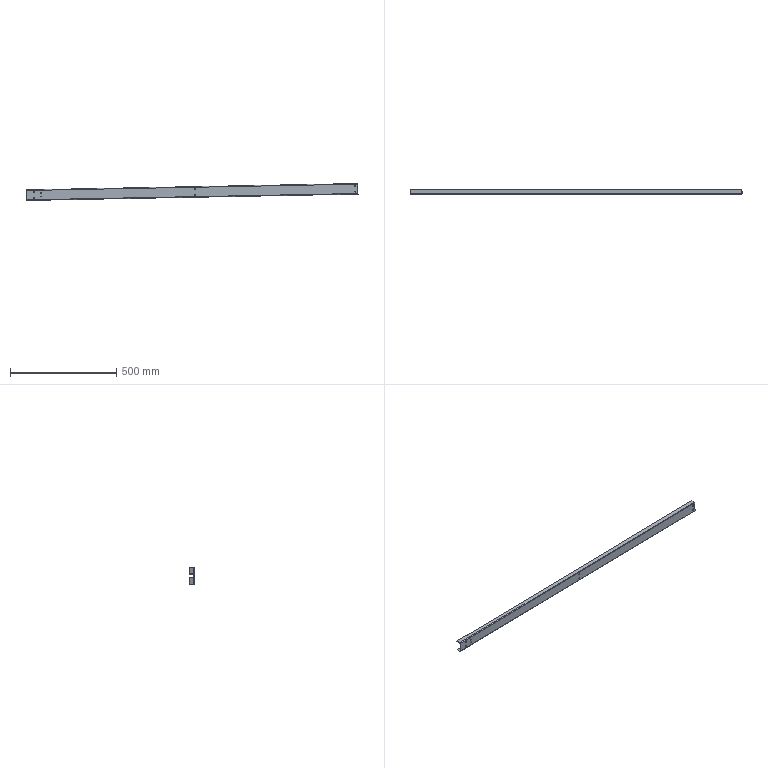Component | SolidWorks | 22DragChainMountingPlate-1 | 1 solid | 38 faces | volume 274965 mm3 | plane 18 | cone 12 | cylinder 8 | commonest cylinder face diameters 4.2 x4 6 x2 2 x2 | material A3 Steel